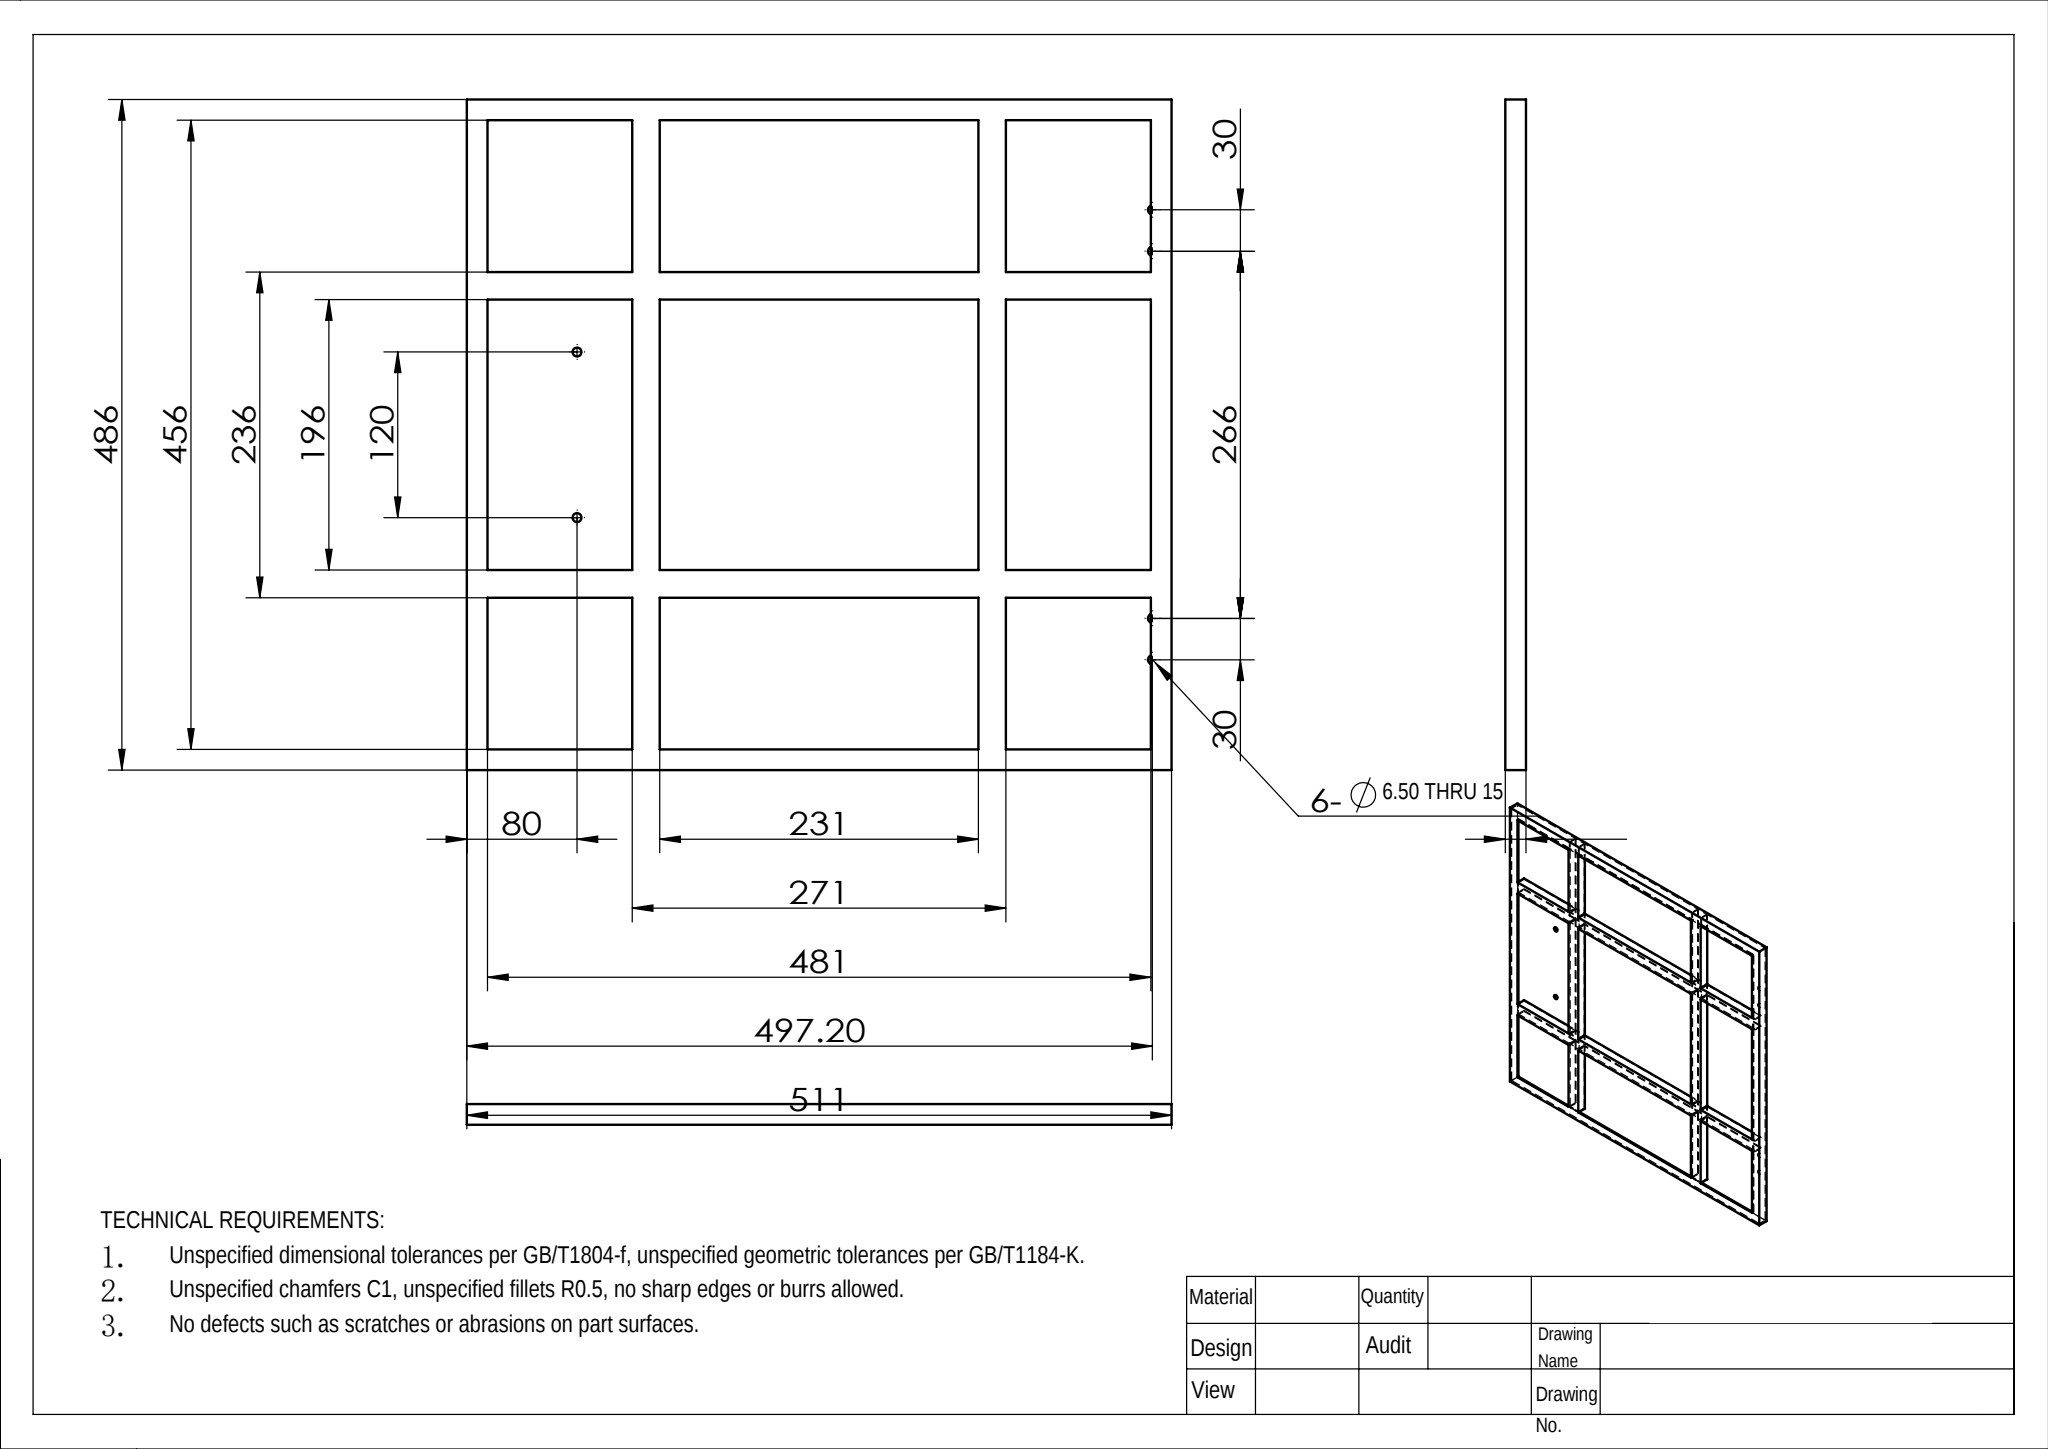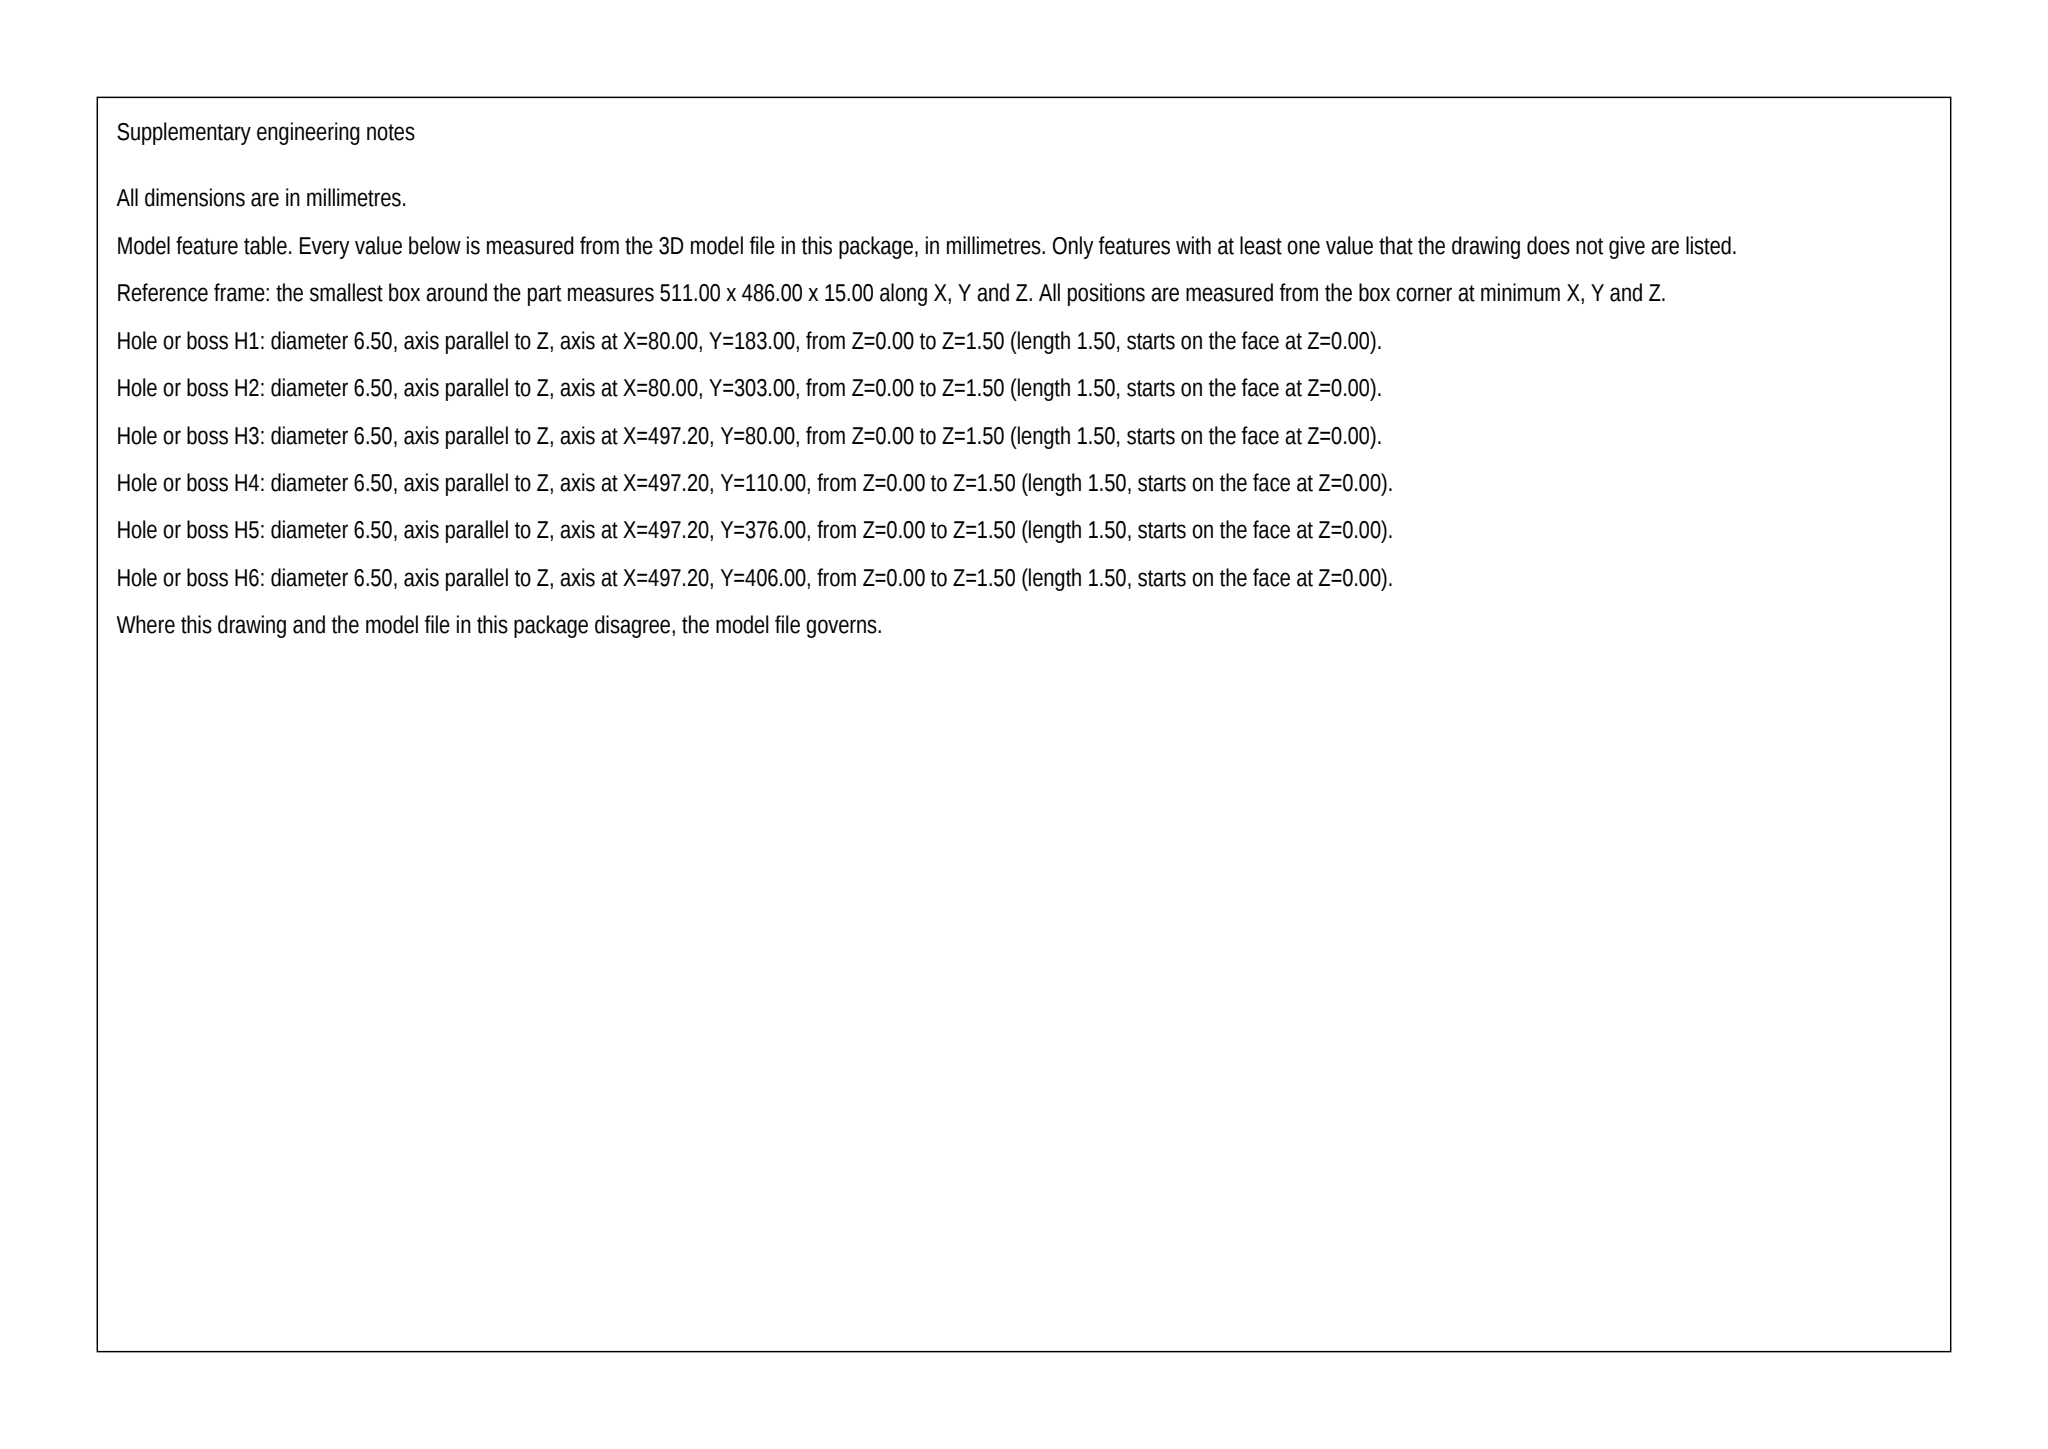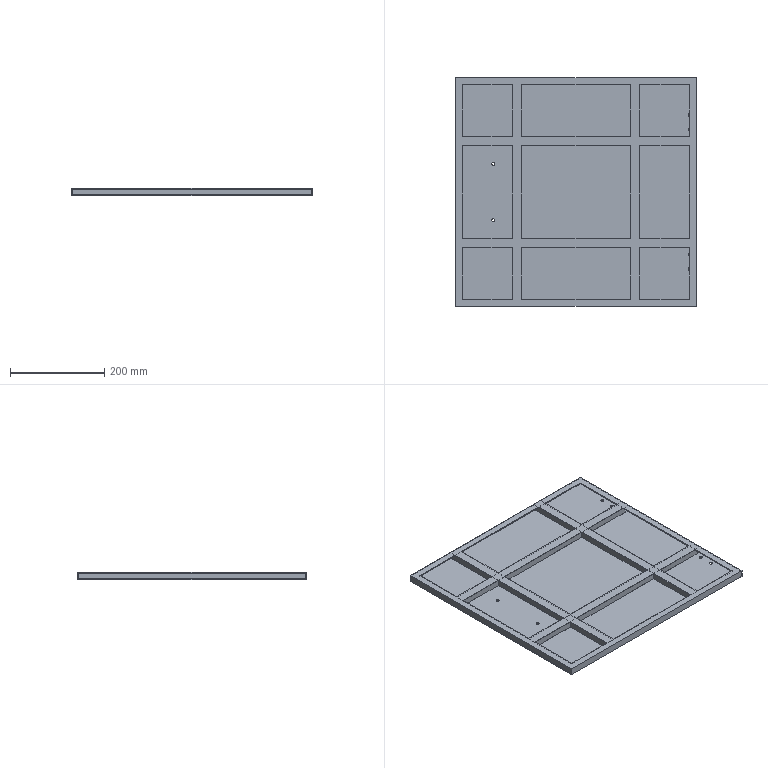Part | SolidWorks | mm | 1 solid | 191 faces | box 511 x 486 x 15 mm | volume 575104 mm3 | plane 179 | cylinder 12 | commonest cylinder face diameters 6.5 x12